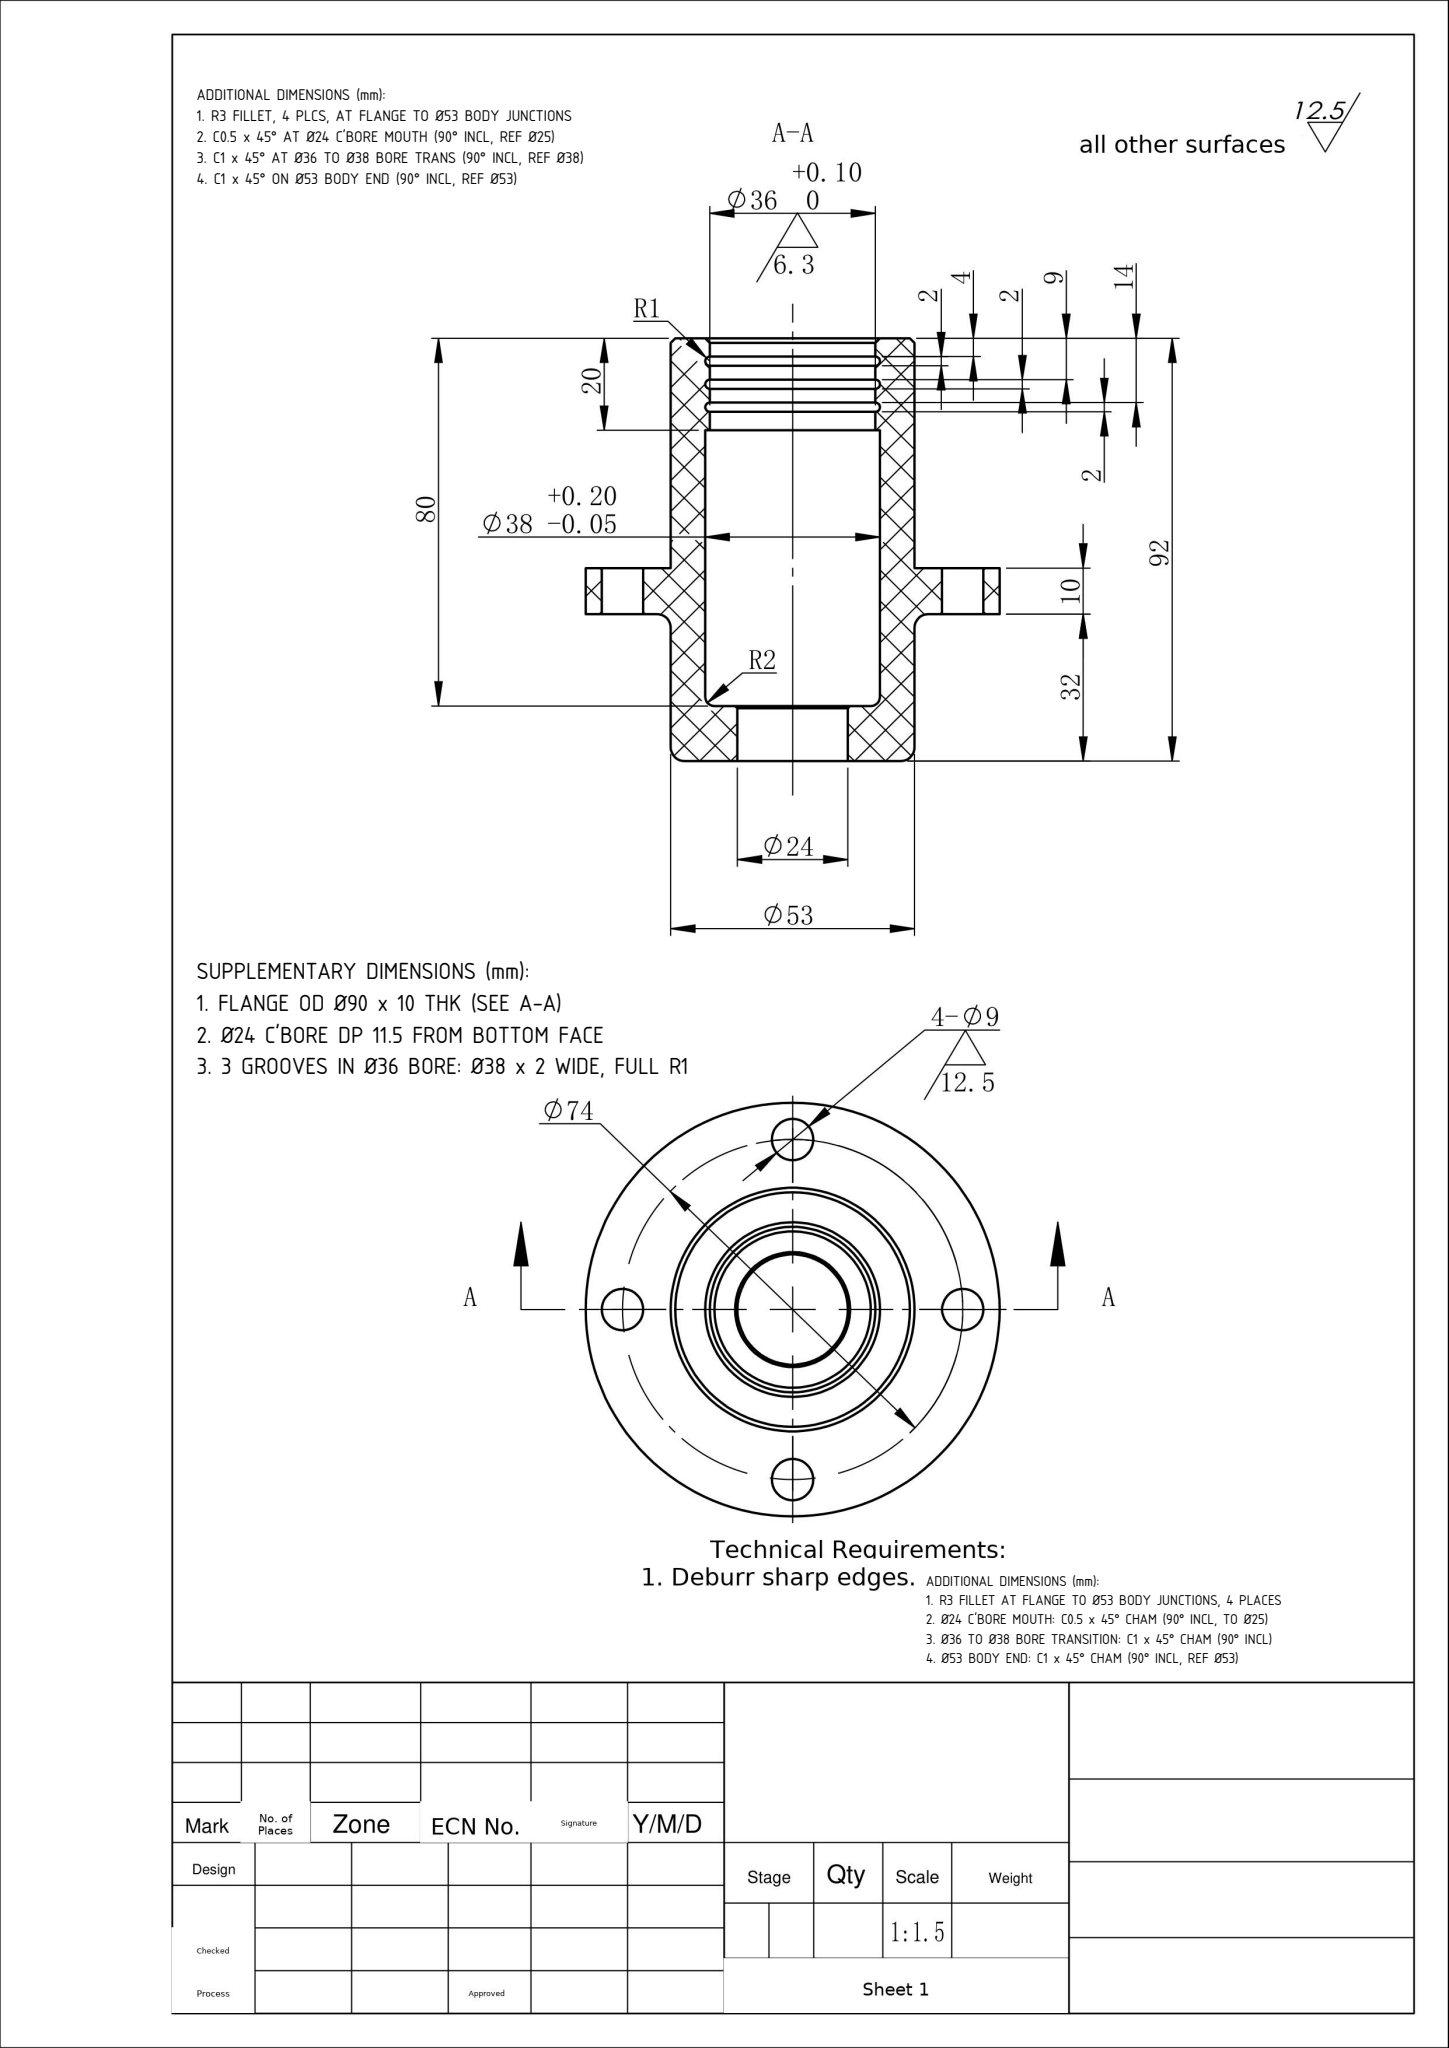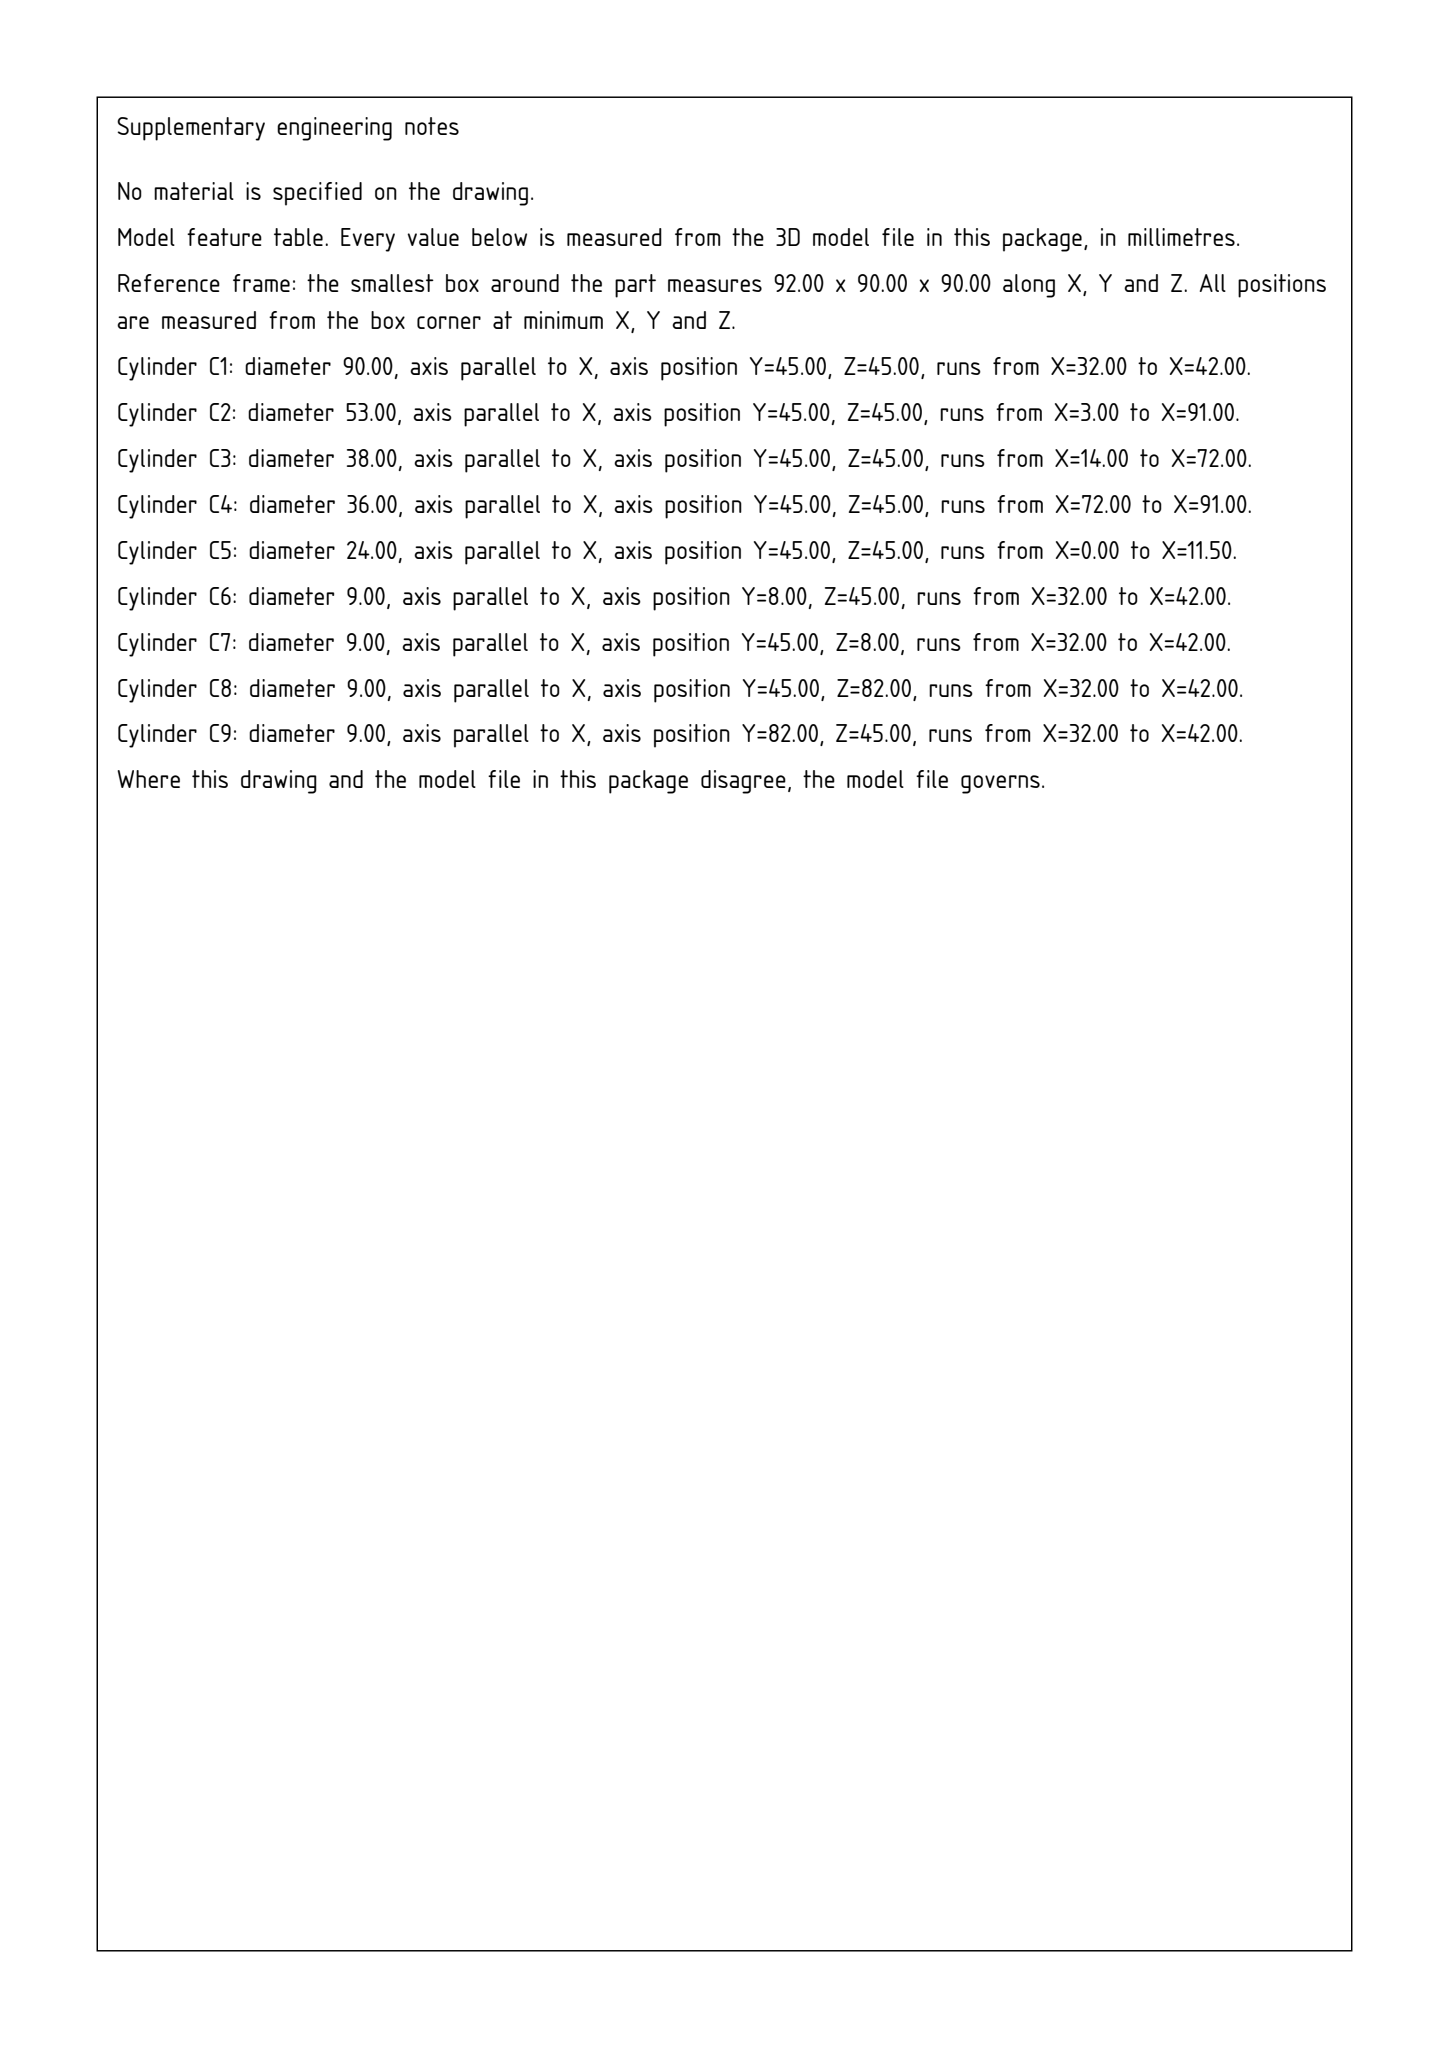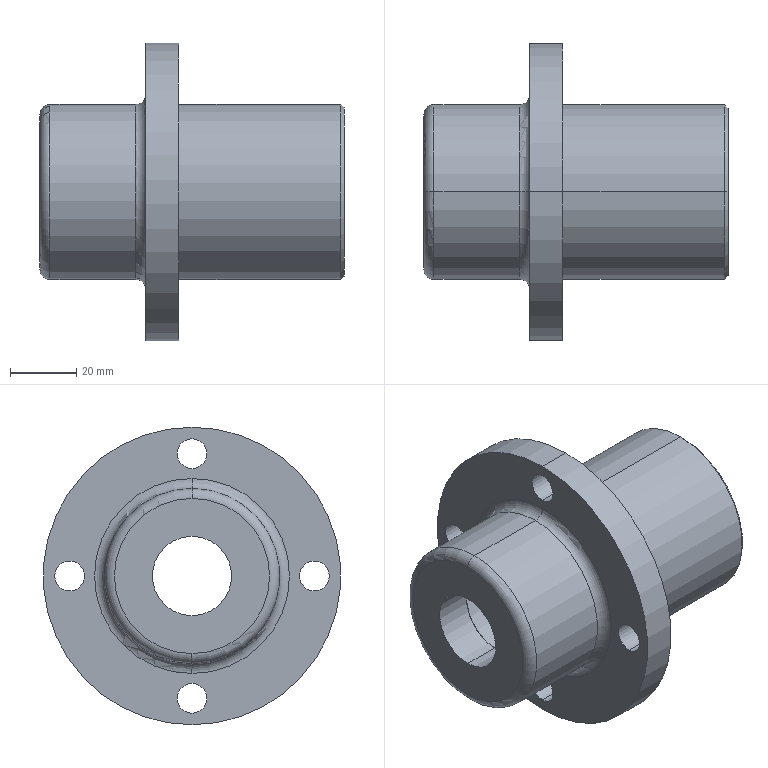Part | SolidWorks | mm | 1 solid | 50 faces | box 92 x 90 x 90 mm | volume 147568 mm3 | cylinder 26 | torus 12 | cone 6 | plane 6 | commonest cylinder face diameters 9 x8 36 x8 53 x4 38 x2 24 x2 90 x2
build123d program:
from build123d import *

# Parameters (mm, degrees)
CHAMFER1_SIZE      = 1
CHAMFER2_SIZE      = 0.5
SKETCH2_R          = 4.5
CUT_EXTRUDE1_DEPTH = 20
CIRPATTERN1_COUNT  = 4


with BuildPart() as part:
    # Sketch1 → Revolve1 (revolve)
    with BuildSketch(Plane.XY, mode=Mode.PRIVATE) as revolve1_sk:
        with BuildLine():
            Line((3, 26.5), (29, 26.5))
            ThreePointArc((29, 26.5), (31.121, 27.379), (32, 29.5))
            Line((32, 29.5), (32, 45))
            Line((32, 45), (42, 45))
            Line((42, 45), (42, 26.5))
            Line((42, 26.5), (92, 26.5))
            Line((92, 26.5), (92, 18))
            Line((92, 18), (88, 18))
            ThreePointArc((88, 18), (87, 19), (86, 18))
            Line((86, 18), (83, 18))
            ThreePointArc((83, 18), (82, 19), (81, 18))
            Line((81, 18), (78, 18))
            ThreePointArc((78, 18), (77, 19), (76, 18))
            Line((76, 18), (72, 18))
            Line((72, 18), (72, 19))
            Line((72, 19), (14, 19))
            ThreePointArc((14, 19), (12.586, 18.414), (12, 17))
            Line((12, 17), (12, 12))
            Line((12, 12), (0, 12))
            Line((0, 12), (0, 23.5))
            ThreePointArc((0, 23.5), (0.8787, 25.621), (3, 26.5))
        make_face()
    revolve(revolve1_sk.sketch.rotate(Axis((0, 0, 0), (1, 0, 0)), 90), axis=Axis((0, 0, 0), (1, 0, 0)))

    # Chamfer1
    chamfer1_edges = [part.edges().sort_by_distance(p)[0] for p in [
        (92, 0, -26.5),
        (92, 0, -18),
    ]]
    chamfer(chamfer1_edges, length=CHAMFER1_SIZE)

    # Chamfer2
    chamfer2_edges = [part.edges().sort_by_distance(p)[0] for p in [
        (12, 0, -12),
    ]]
    chamfer(chamfer2_edges, length=CHAMFER2_SIZE)

    # Sketch2 → Cut-Extrude1 (cut)
    with BuildSketch(Plane.ZY.offset(-32)):
        with Locations((0, 37)):
            Circle(SKETCH2_R)
    cut_extrude1 = extrude(amount=-CUT_EXTRUDE1_DEPTH, mode=Mode.SUBTRACT)

    # CirPattern1: Cut-Extrude1 ×4 about axis
    cirpattern1_axis = Axis((0, 0, 0), (1, 0, 0))
    for i in range(1, CIRPATTERN1_COUNT):
        add(cut_extrude1.rotate(cirpattern1_axis, i * 360 / CIRPATTERN1_COUNT), mode=Mode.SUBTRACT)


solid = part.part